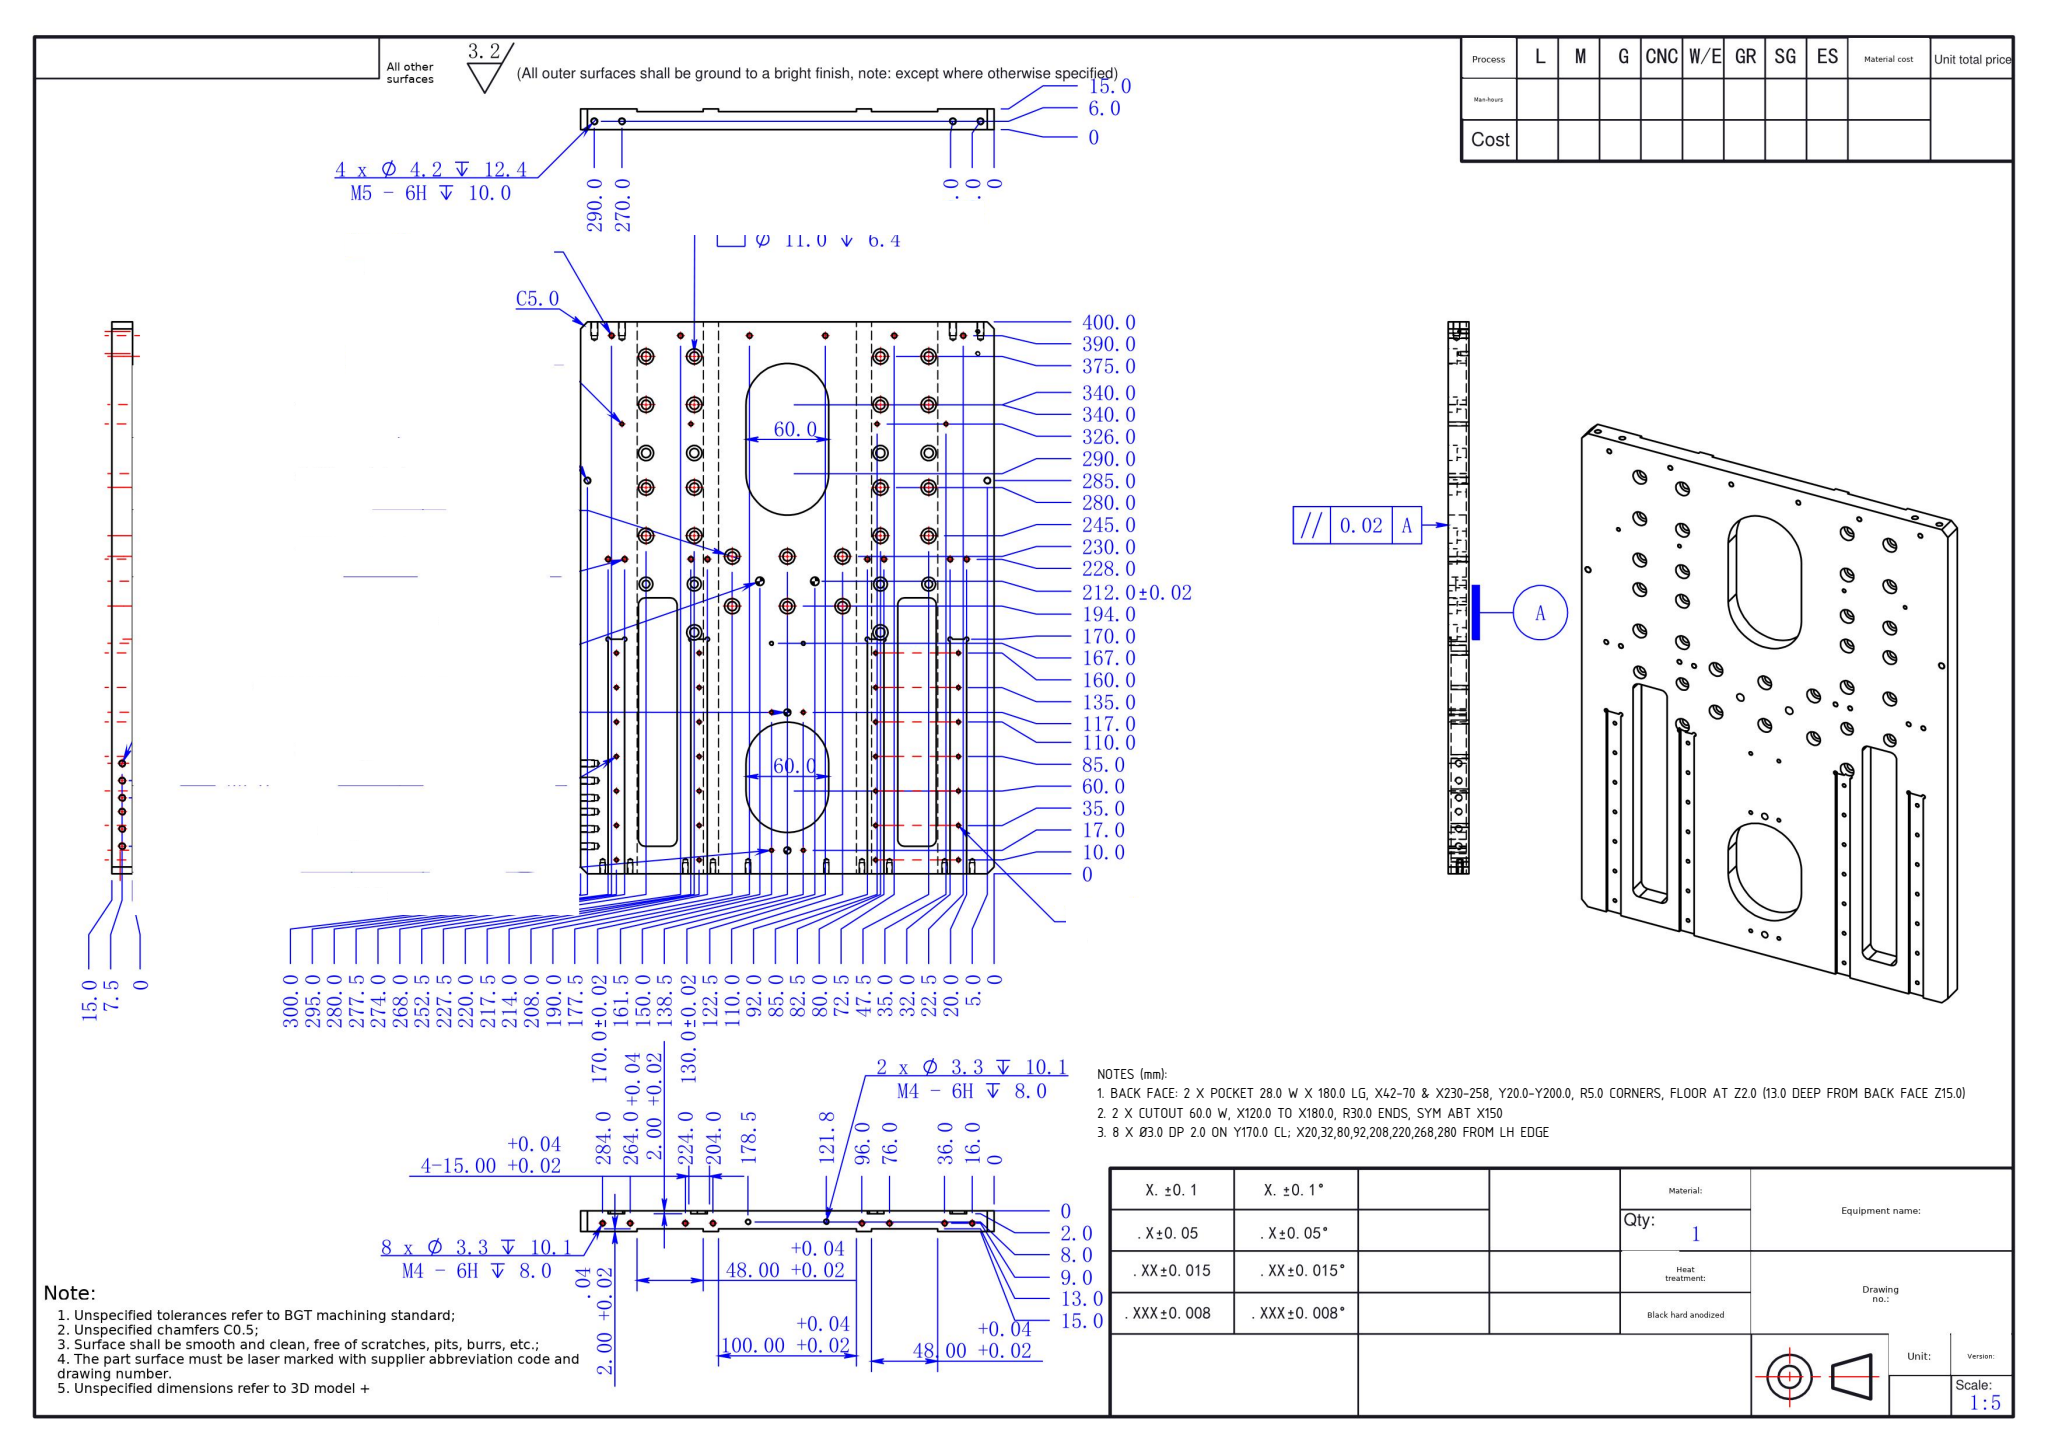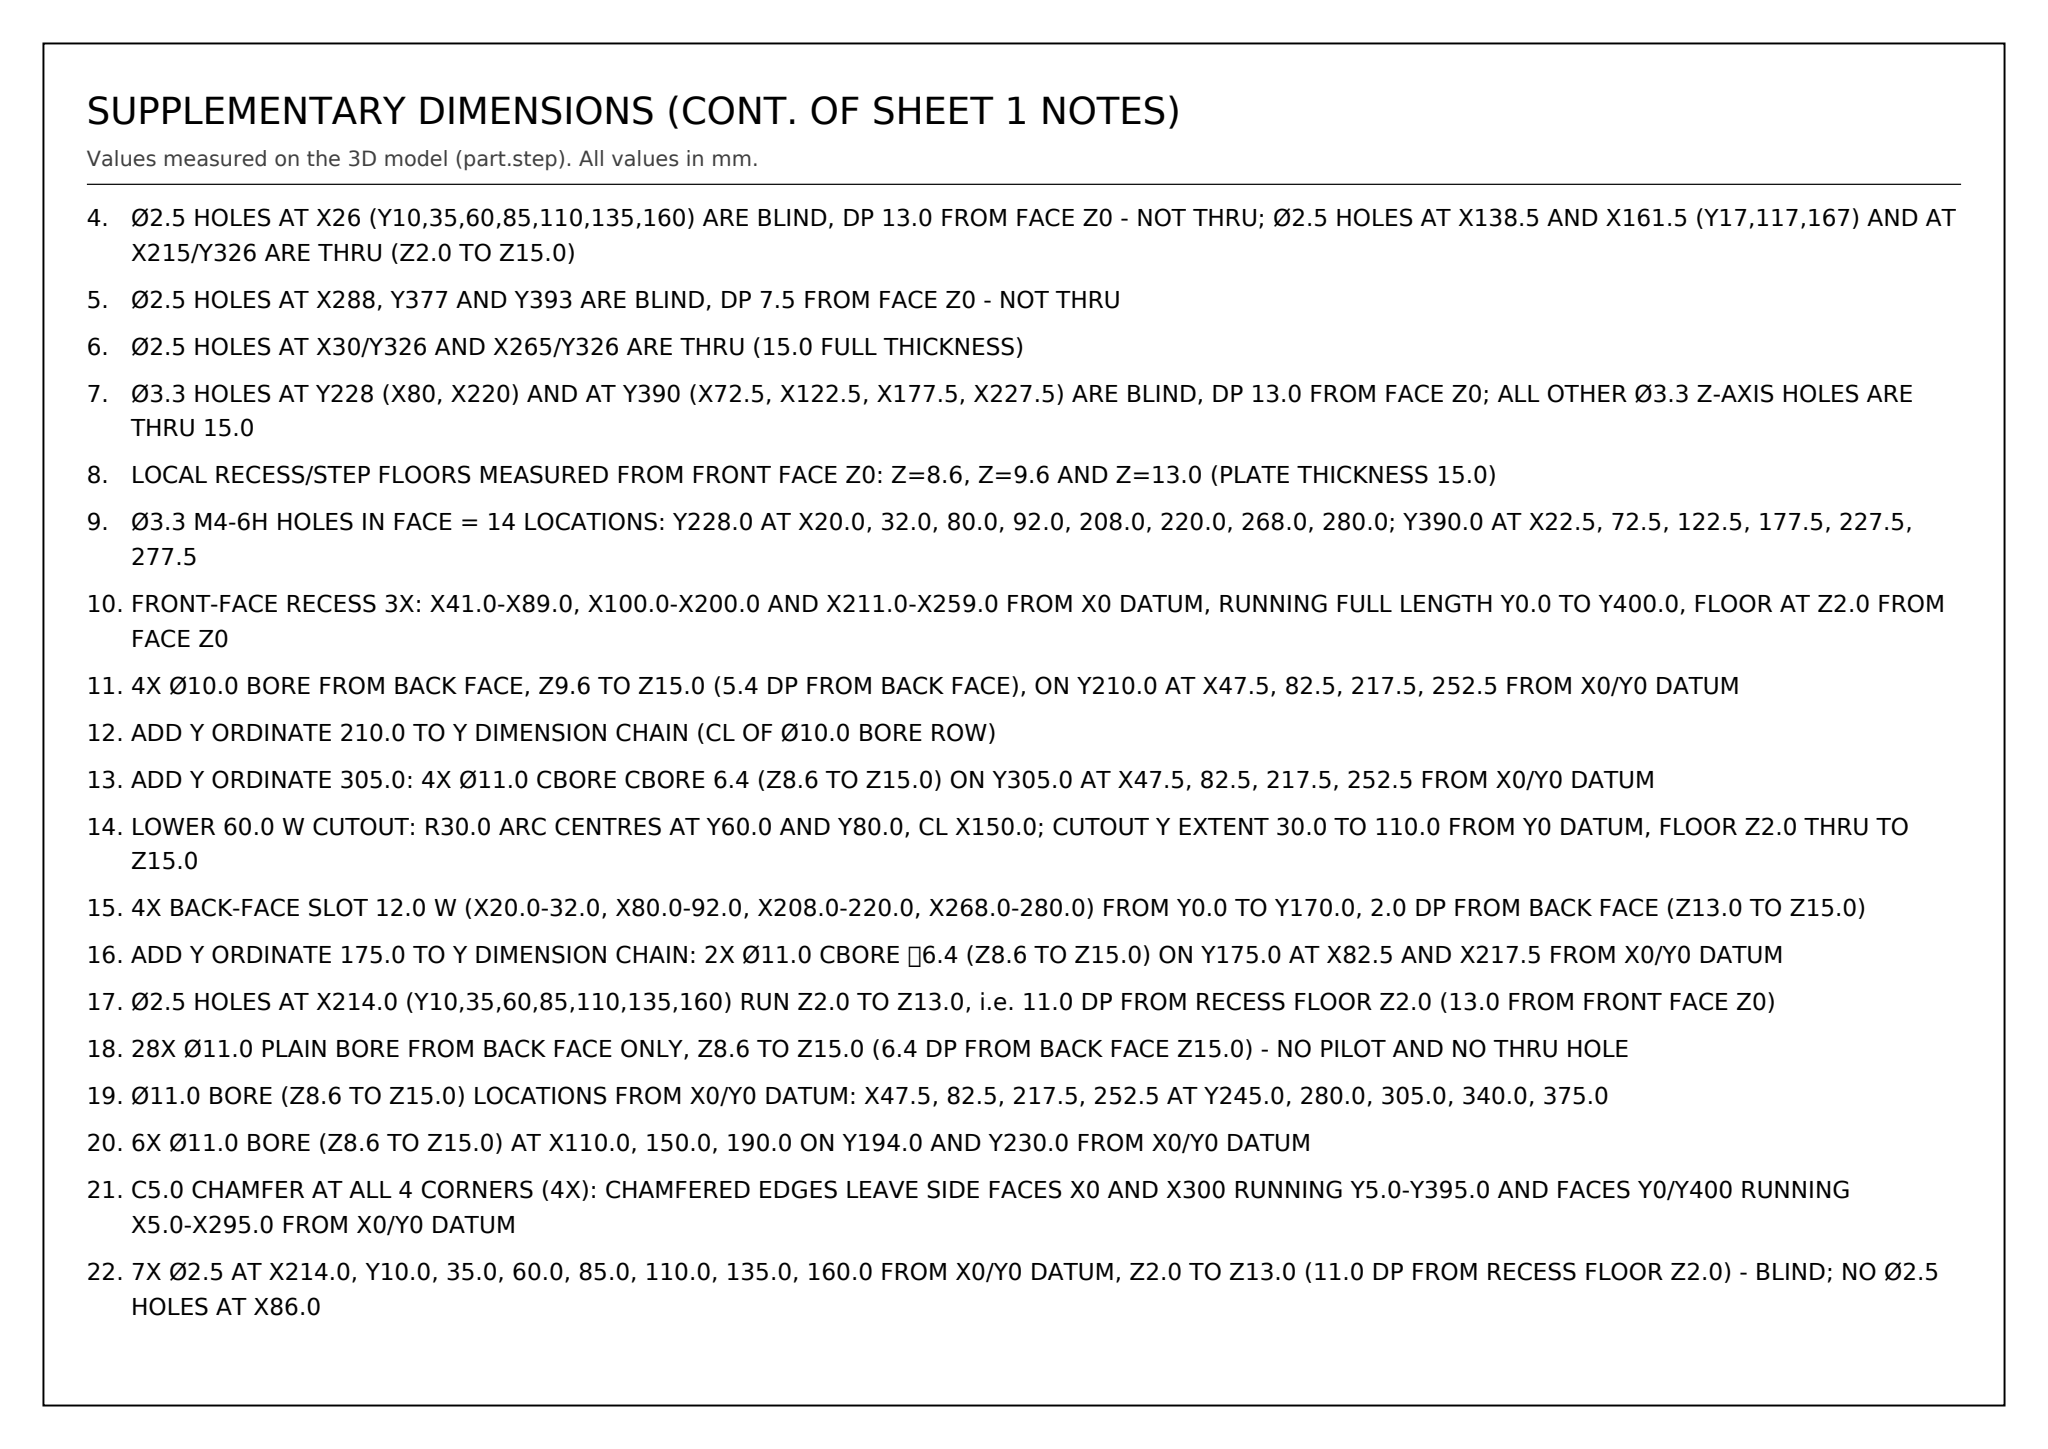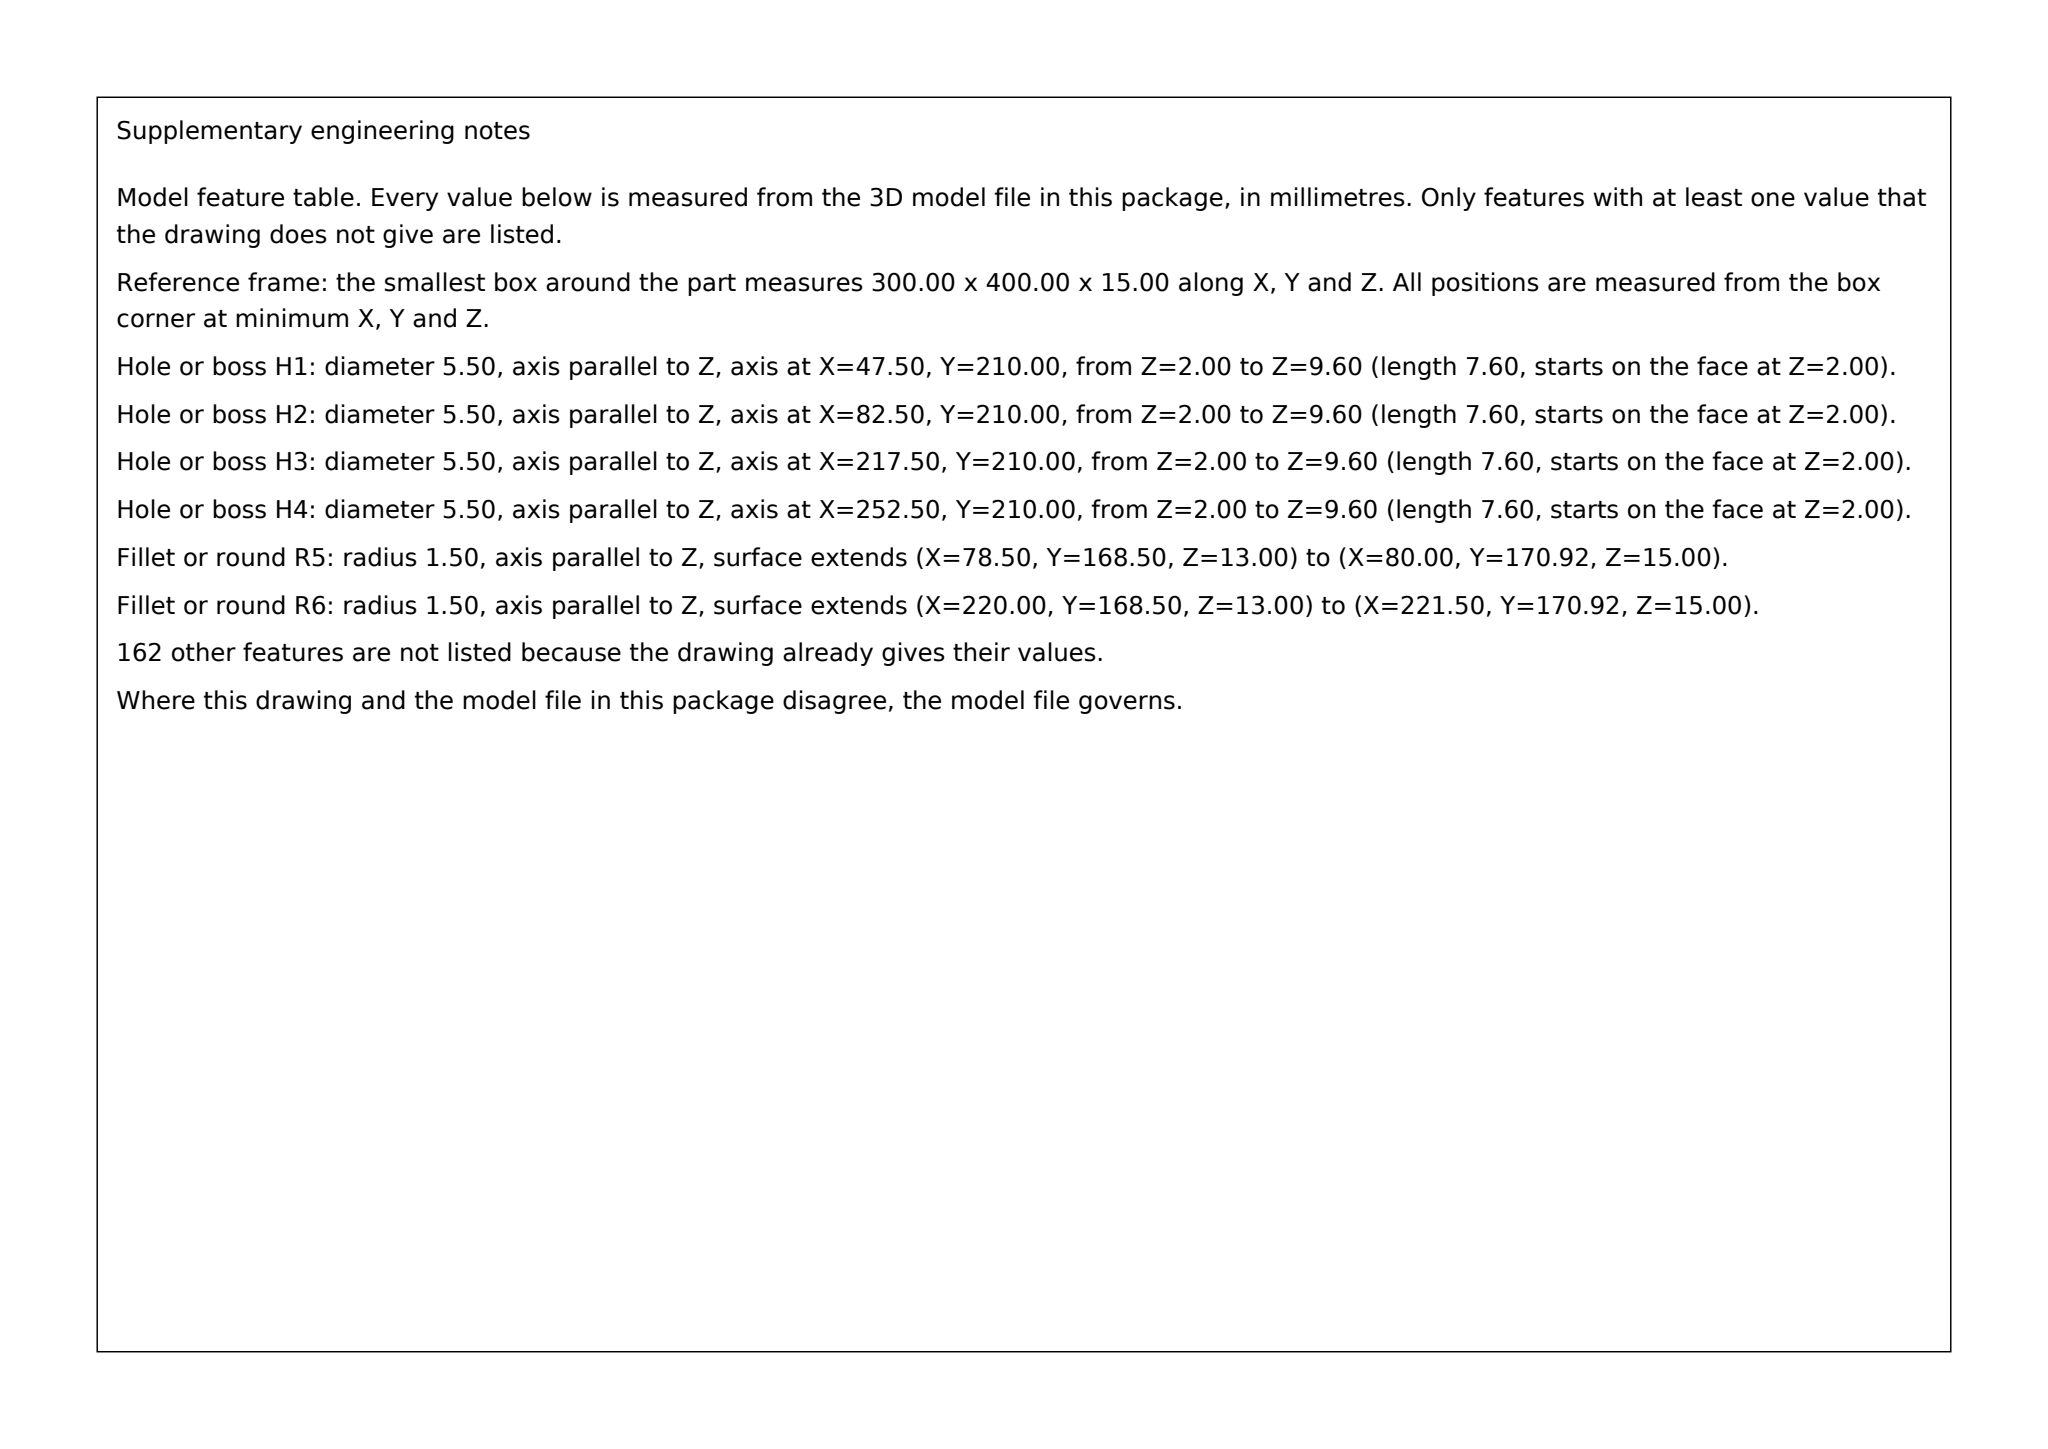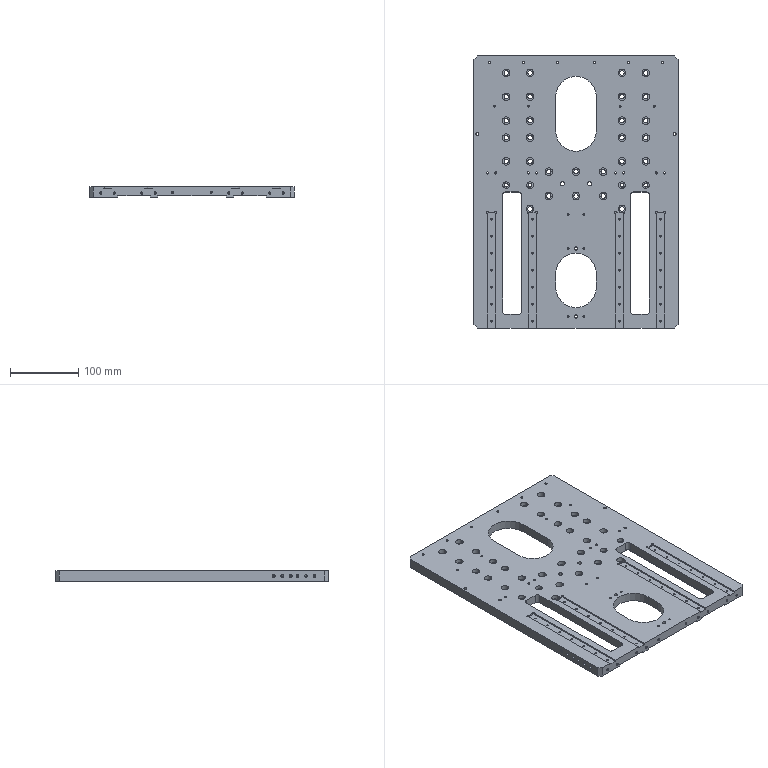Part | SolidWorks | mm | 1 solid | 438 faces | box 300 x 400 x 15 mm | volume 1333290 mm3 | cylinder 312 | plane 82 | cone 44 | commonest cylinder face diameters 2.5 x80 11 x56 6.6 x56 3.3 x48 4.2 x24 10 x16 3 x12 5.5 x8
Drawing notes:
BACK FACE: 2 X POCKET 28.0 W X 180.0 LG, X42-70 & X230-258, Y20.0-Y200.0, R5.0 CORNERS, FLOOR AT Z2.0 (13.0 DEEP FROM BACK FACE Z15.0) | from the solid: x-planes at 42.0, 70.0, 230.0, 258.0 (y 25.0-195.0, z 2.0-15.0) and y-planes at 20.0 & 200.0 (x 47-65 and 235-253, z 2.0-15.0); corner arcs are dia 10.0 (= R5.0) at (47,25),(47,195),(65,25),(65,195),(235,25),(235,195),(253,25),(253,195), z 2.0 to 15.0
2 X CUTOUT 60.0 W, X120.0 TO X180.0, R30.0 ENDS, SYM ABT X150 | from the solid: axis planes x=120.0 (2) and x=180.0 (2) = flats of two 60 wide cutouts, sym about X150
8 X Ø3.0 DP 2.0 ON Y170.0 CL; X20,32,80,92,208,220,268,280 FROM LH EDGE | from the solid: cylinders dia 3.0, axis z, y=170, len 2.0 at x=20,32,80,92,208,220,268,280 (8 holes)
Ø2.5 HOLES AT X26 (Y10,35,60,85,110,135,160) ARE BLIND, DP 13.0 FROM FACE Z0 - NOT THRU; Ø2.5 HOLES AT X138.5 AND X161.5 (Y17,117,167) AND AT X215/Y326 ARE THRU (Z2.0 TO Z15.0) | from the solid: hole/bore 2.5 z at [26.0,10/35/60/85/110/135/160] from 0.0 to 13.0 (blind); hole/bore 2.5 z at [138.5,17/117/167] and [161.5,17/117/167] from 2.0 to 15.0 (thru); hole/bore 2.5 z at [215.0,326.0] from 2.0 to 15.0 (thru)
Ø2.5 HOLES AT X288, Y377 AND Y393 ARE BLIND, DP 7.5 FROM FACE Z0 - NOT THRU | from the solid: cylinders [2.5,'z',[288.0,377.0/393.0,null],7.5,2]
Ø2.5 HOLES AT X30/Y326 AND X265/Y326 ARE THRU (15.0 FULL THICKNESS) | from the solid: cylinders [2.5,'z',[30.0/265.0,326.0,null],15.0,2]
Ø3.3 HOLES AT Y228 (X80, X220) AND AT Y390 (X72.5, X122.5, X177.5, X227.5) ARE BLIND, DP 13.0 FROM FACE Z0; ALL OTHER Ø3.3 Z-AXIS HOLES ARE THRU 15.0 | from the solid: cylinders [3.3,'z',...,13.0] vs [3.3,'z',...,15.0]
LOCAL RECESS/STEP FLOORS MEASURED FROM FRONT FACE Z0: Z=8.6, Z=9.6 AND Z=13.0 (PLATE THICKNESS 15.0) | from the solid: axis_planes ['z',8.6,28], ['z',9.6,4], ['z',13.0,4], ['z',15.0,1]
Ø3.3 M4-6H HOLES IN FACE = 14 LOCATIONS: Y228.0 AT X20.0, 32.0, 80.0, 92.0, 208.0, 220.0, 268.0, 280.0; Y390.0 AT X22.5, 72.5, 122.5, 177.5, 227.5, 277.5 | from the solid: cylinders dia 3.3 axis z, [x,y] positions
FRONT-FACE RECESS 3X: X41.0-X89.0, X100.0-X200.0 AND X211.0-X259.0 FROM X0 DATUM, RUNNING FULL LENGTH Y0.0 TO Y400.0, FLOOR AT Z2.0 FROM FACE Z0 | from the solid: x-planes at 41.0, 89.0, 100.0, 200.0, 211.0 and 259.0 each with extent y [0.0,400.0], z [0.0,2.0], area 800; holes at X138.5/X161.5 and X214 start at z 2.0 while holes at X26 start at z 0.0
4X Ø10.0 BORE FROM BACK FACE, Z9.6 TO Z15.0 (5.4 DP FROM BACK FACE), ON Y210.0 AT X47.5, 82.5, 217.5, 252.5 FROM X0/Y0 DATUM | from the solid: cylinders: hole/bore dia 10.0 axis z at (47.5,210),(82.5,210),(217.5,210),(252.5,210), from 9.6 to 15.0
ADD Y ORDINATE 210.0 TO Y DIMENSION CHAIN (CL OF Ø10.0 BORE ROW) | from the solid: cylinders: hole/bore dia 10.0 axis z at y=210.0 (X47.5, 82.5, 217.5, 252.5)
ADD Y ORDINATE 305.0: 4X Ø11.0 CBORE CBORE 6.4 (Z8.6 TO Z15.0) ON Y305.0 AT X47.5, 82.5, 217.5, 252.5 FROM X0/Y0 DATUM | from the solid: cylinders: hole/bore dia 11.0 axis z at (47.5,305),(82.5,305),(217.5,305),(252.5,305), from 8.6 to 15.0
LOWER 60.0 W CUTOUT: R30.0 ARC CENTRES AT Y60.0 AND Y80.0, CL X150.0; CUTOUT Y EXTENT 30.0 TO 110.0 FROM Y0 DATUM, FLOOR Z2.0 THRU TO Z15.0 | from the solid: cylinders: concave arc dia 60.0 axis z at (150,60) and (150,80), from 2.0 to 15.0, 180 deg each
4X BACK-FACE SLOT 12.0 W (X20.0-32.0, X80.0-92.0, X208.0-220.0, X268.0-280.0) FROM Y0.0 TO Y170.0, 2.0 DP FROM BACK FACE (Z13.0 TO Z15.0) | from the solid: axis_planes: x=20/32/80/92/208/220/268/280 with y extent [0.0,168.5], z extent [13.0,15.0]
ADD Y ORDINATE 175.0 TO Y DIMENSION CHAIN: 2X Ø11.0 CBORE ⍄6.4 (Z8.6 TO Z15.0) ON Y175.0 AT X82.5 AND X217.5 FROM X0/Y0 DATUM | from the solid: cylinders: hole/bore dia 11.0, axis z at (82.5,175.0) and (217.5,175.0), from Z8.6 to Z15.0
Ø2.5 HOLES AT X214.0 (Y10,35,60,85,110,135,160) RUN Z2.0 TO Z13.0, i.e. 11.0 DP FROM RECESS FLOOR Z2.0 (13.0 FROM FRONT FACE Z0) | from the solid: cylinders: hole/bore dia 2.5 axis z at [214.0,10.0 ...160.0], from 2.0 to 13.0
28X Ø11.0 PLAIN BORE FROM BACK FACE ONLY, Z8.6 TO Z15.0 (6.4 DP FROM BACK FACE Z15.0) - NO PILOT AND NO THRU HOLE | from the solid: cylinders kind hole/bore dia 11.0 axis z, from 8.6 to 15.0 (28 occurrences)
Ø11.0 BORE (Z8.6 TO Z15.0) LOCATIONS FROM X0/Y0 DATUM: X47.5, 82.5, 217.5, 252.5 AT Y245.0, 280.0, 305.0, 340.0, 375.0 | from the solid: cylinders dia 11.0 axis z at (47.5/82.5/217.5/252.5, 245/280/305/340/375), from 8.6 to 15.0
6X Ø11.0 BORE (Z8.6 TO Z15.0) AT X110.0, 150.0, 190.0 ON Y194.0 AND Y230.0 FROM X0/Y0 DATUM | from the solid: cylinders dia 11.0 axis z at [110/150/190, 194.0] and [110/150/190, 230.0], from 8.6 to 15.0
C5.0 CHAMFER AT ALL 4 CORNERS (4X): CHAMFERED EDGES LEAVE SIDE FACES X0 AND X300 RUNNING Y5.0-Y395.0 AND FACES Y0/Y400 RUNNING X5.0-X295.0 FROM X0/Y0 DATUM | from the solid: axis_planes: x=0.0 extent y[5.0,395.0]; x=300.0 extent y[5.0,395.0]; y=0.0 extent x[5.0,295.0] (bbox 300.0 x 400.0 x 15.0)
7X Ø2.5 AT X214.0, Y10.0, 35.0, 60.0, 85.0, 110.0, 135.0, 160.0 FROM X0/Y0 DATUM, Z2.0 TO Z13.0 (11.0 DP FROM RECESS FLOOR Z2.0) - BLIND; NO Ø2.5 HOLES AT X86.0 | from the solid: cylinders hole/bore Ø2.5 z-axis at (214.0, 10/35/60/85/110/135/160) from 2.0 to 13.0; no Ø2.5 cylinder at X86.0 in model
build123d program:
from build123d import *

# Parameters (mm, degrees)
SKETCH1_W                                       = 300
SKETCH1_H                                       = 285
BOSS_EXTRUDE1_DEPTH                             = 15
SKETCH2_W                                       = 300
SKETCH2_H                                       = 15
BOSS_EXTRUDE2_DEPTH                             = 115
CHAMFER2_SIZE                                   = 5
SKETCH4_W                                       = 12
SKETCH4_H                                       = 2
CUT_EXTRUDE2_DEPTH                              = 170
SKETCH5_R                                       = 1.5
CUT_EXTRUDE3_DEPTH                              = 2
SKETCH6_W                                       = 48
SKETCH6_H                                       = 2
CUT_EXTRUDE4_DEPTH                              = 428.463
SKETCH7_W                                       = 100
SKETCH7_H                                       = 2
CUT_EXTRUDE5_DEPTH                              = 428.463
SKETCH8_R                                       = 30
CUT_EXTRUDE6_DEPTH                              = 299.287
M6_HEX_SOCKET_HEAD_CAP_SCREW_CBORE1_D           = 6.6
M6_HEX_SOCKET_HEAD_CAP_SCREW_CBORE1_CBORE_D     = 11
M6_HEX_SOCKET_HEAD_CAP_SCREW_CBORE1_CBORE_DEPTH = 6.4
M6_HEX_SOCKET_HEAD_CAP_SCREW_CBORE2_D           = 6.6
M6_HEX_SOCKET_HEAD_CAP_SCREW_CBORE2_CBORE_D     = 11
M6_HEX_SOCKET_HEAD_CAP_SCREW_CBORE2_CBORE_DEPTH = 6.4
M4_TAPPED_HOLE1_D                               = 3.3
M4_TAPPED_HOLE1_DEPTH                           = 10.1
M4_TAPPED_HOLE1_TIP                             = 0.9914
SIZE_MM_DOWEL_PIN_HOLE_1_D                      = 6
CUT_EXTRUDE7_DEPTH                              = 299.381
CUT_EXTRUDE8_DEPTH                              = 299.381
M3_TAPPED_HOLE1_D                               = 2.5
M3_TAPPED_HOLE2_D                               = 2.5
M3_TAPPED_HOLE2_DEPTH                           = 7.5
M3_TAPPED_HOLE2_TIP                             = 0.7511
M4_TAPPED_HOLE3_D                               = 3.3
M3_TAPPED_HOLE3_D                               = 2.5
LPATTERN1_COUNT                                 = 2
LPATTERN1_PITCH                                 = 60
MIRROR3_COPY_1_D                                = 2.5
M4_TAPPED_HOLE2_D                               = 3.3
M3_TAPPED_HOLE4_D                               = 2.5
SIZE_MM_DOWEL_PIN_HOLE_2_D                      = 5
SKETCH35_W                                      = 28
SKETCH35_H                                      = 180
CUT_EXTRUDE9_DEPTH                              = 299.381
FILLET2_R                                       = 5
M5_TAPPED_HOLE1_D                               = 4.2
M5_TAPPED_HOLE1_DEPTH                           = 12.4
M5_TAPPED_HOLE1_TIP                             = 1.262
M5_HEX_SOCKET_HEAD_CAP_SCREW_CBORE2_D           = 5.5
M5_HEX_SOCKET_HEAD_CAP_SCREW_CBORE2_CBORE_D     = 10
M5_HEX_SOCKET_HEAD_CAP_SCREW_CBORE2_CBORE_DEPTH = 5.4
M6_HEX_SOCKET_HEAD_CAP_SCREW_CBORE3_D           = 6.6
M6_HEX_SOCKET_HEAD_CAP_SCREW_CBORE3_CBORE_D     = 11
M6_HEX_SOCKET_HEAD_CAP_SCREW_CBORE3_CBORE_DEPTH = 6.4
M4_TAPPED_HOLE4_D                               = 3.3
M4_TAPPED_HOLE4_DEPTH                           = 10.1
M4_TAPPED_HOLE4_TIP                             = 0.9914
M5_TAPPED_HOLE2_D                               = 4.2
M5_TAPPED_HOLE2_DEPTH                           = 12.4
M5_TAPPED_HOLE2_TIP                             = 1.262
M5_TAPPED_HOLE3_D                               = 4.2


with BuildPart() as part:
    # Sketch1 → Boss-Extrude1 (new body)
    with BuildSketch(Plane.XY):
        Rectangle(SKETCH1_W, SKETCH1_H)
    extrude(amount=BOSS_EXTRUDE1_DEPTH)

    # Sketch2 → Boss-Extrude2 (add)
    with BuildSketch(Plane(origin=(0, 142.5, 0), x_dir=(1, 0, 0), z_dir=(0, 1, 0))):
        with Locations((0, -7.5)):
            Rectangle(SKETCH2_W, SKETCH2_H)
    extrude(amount=BOSS_EXTRUDE2_DEPTH)

    # Chamfer2
    chamfer2_edges = [part.edges().sort_by_distance(p)[0] for p in [
        (150, 257.5, 7.5),
        (-150, 257.5, 7.5),
        (150, -142.5, 7.5),
        (-150, -142.5, 7.5),
    ]]
    chamfer(chamfer2_edges, length=CHAMFER2_SIZE)

    # Sketch4 → Cut-Extrude2 (cut)
    with BuildSketch(Plane.XZ.offset(142.5)):
        with Locations((-124, 14)):
            Rectangle(SKETCH4_W, SKETCH4_H)
        with Locations((-64, 14)):
            Rectangle(SKETCH4_W, SKETCH4_H)
    cut_extrude2 = extrude(amount=-CUT_EXTRUDE2_DEPTH, mode=Mode.SUBTRACT)

    # Sketch5 → Cut-Extrude3 (cut)
    with BuildSketch(Plane.XY.offset(15)):
        with Locations((-130, 27.5)):
            Circle(SKETCH5_R)
        with Locations((-118, 27.5)):
            Circle(SKETCH5_R)
        with Locations((-70, 27.5)):
            Circle(SKETCH5_R)
        with Locations((-58, 27.5)):
            Circle(SKETCH5_R)
    cut_extrude3 = extrude(amount=-CUT_EXTRUDE3_DEPTH, mode=Mode.SUBTRACT)

    # Mirror1: Cut-Extrude2, Cut-Extrude3 across plane
    add(cut_extrude2.mirror(Plane.ZY), mode=Mode.SUBTRACT)
    add(cut_extrude3.mirror(Plane.ZY), mode=Mode.SUBTRACT)

    # Sketch6 → Cut-Extrude4 (cut, through all)
    with BuildSketch(Plane(origin=(0, 257.5, 0), x_dir=(1, 0, 0), z_dir=(0, 1, 0))):
        with Locations((85, -1)):
            Rectangle(SKETCH6_W, SKETCH6_H)
        with Locations((-85, -1)):
            Rectangle(SKETCH6_W, SKETCH6_H)
    extrude(amount=-CUT_EXTRUDE4_DEPTH, mode=Mode.SUBTRACT)

    # Sketch7 → Cut-Extrude5 (cut, through all)
    with BuildSketch(Plane(origin=(0, 257.5, 0), x_dir=(1, 0, 0), z_dir=(0, 1, 0))):
        with Locations((0, -1)):
            Rectangle(SKETCH7_W, SKETCH7_H)
    extrude(amount=-CUT_EXTRUDE5_DEPTH, mode=Mode.SUBTRACT)

    # Sketch8 → Cut-Extrude6 (cut, through all)
    with BuildSketch(Plane(origin=(0, 0, 2), x_dir=(-1, 0, 0), z_dir=(0, 0, -1))):
        with Locations((0, 197.5)):
            Circle(SKETCH8_R)
        with Locations((0, -82.5)):
            Circle(SKETCH8_R)
    extrude(amount=-CUT_EXTRUDE6_DEPTH, mode=Mode.SUBTRACT)

    # M6 Hex Socket Head Cap Screw CBORE1 (through all)
    with Locations(Plane.XY.offset(15)):
        with Locations((-40, 87.5), (40, 87.5), (-40, 51.5), (40, 51.5), (0, 87.5), (0, 51.5)):
            CounterBoreHole(M6_HEX_SOCKET_HEAD_CAP_SCREW_CBORE1_D / 2, M6_HEX_SOCKET_HEAD_CAP_SCREW_CBORE1_CBORE_D / 2, M6_HEX_SOCKET_HEAD_CAP_SCREW_CBORE1_CBORE_DEPTH)

    # M6 Hex Socket Head Cap Screw CBORE2 (through all)
    with Locations(Plane.XY.offset(15)):
        with Locations((102.5, 232.5), (67.5, 232.5), (67.5, 197.5), (102.5, 197.5), (67.5, 137.5), (102.5, 137.5), (67.5, 102.5), (102.5, 102.5)):
            m6_hex_socket_head_cap_screw_cbore2 = CounterBoreHole(M6_HEX_SOCKET_HEAD_CAP_SCREW_CBORE2_D / 2, M6_HEX_SOCKET_HEAD_CAP_SCREW_CBORE2_CBORE_D / 2, M6_HEX_SOCKET_HEAD_CAP_SCREW_CBORE2_CBORE_DEPTH)

    # Mirror2: M6 Hex Socket Head Cap Screw CBORE2 across plane
    add(m6_hex_socket_head_cap_screw_cbore2.mirror(Plane(origin=(0, 0, 0), x_dir=(0, 0, 1), z_dir=(1, 0, 0))), mode=Mode.SUBTRACT)

    # M4 Tapped Hole1
    with Locations(Plane(origin=(0, -142.5, 0), x_dir=(-1, 0, 0), z_dir=(0, -1, 0))):
        with Locations((134, -6), (114, -6), (74, -6), (54, -6), (-54, -6), (-74, -6), (-114, -6), (-134, -6)):
            Hole(M4_TAPPED_HOLE1_D / 2, depth=M4_TAPPED_HOLE1_DEPTH)
            with Locations((0, 0, -(M4_TAPPED_HOLE1_DEPTH + M4_TAPPED_HOLE1_TIP / 2))):  # 118° drill point
                Cone(0, M4_TAPPED_HOLE1_D / 2, M4_TAPPED_HOLE1_TIP, mode=Mode.SUBTRACT)

    # Size mm Dowel Pin Hole 1 (through all)
    with Locations(Plane.XY.offset(15)):
        with Locations((-20, 69.5), (20, 69.5)):
            Hole(SIZE_MM_DOWEL_PIN_HOLE_1_D / 2)

    # Sketch19 → Cut-Extrude7 (cut, through all)
    with BuildSketch(Plane.XY.offset(15)):
        with BuildLine():
            Line((30, 197.5), (30, 147.5))
            ThreePointArc((30, 147.5), (0, 117.5), (-30, 147.5))
            Line((-30, 147.5), (-30, 197.5))
            ThreePointArc((-30, 197.5), (0, 227.5), (30, 197.5))
        make_face()
    extrude(amount=-CUT_EXTRUDE7_DEPTH, mode=Mode.SUBTRACT)

    # Sketch20 → Cut-Extrude8 (cut, through all)
    with BuildSketch(Plane.XY.offset(15)):
        with BuildLine():
            Line((-30, -82.5), (-30, -62.5))
            ThreePointArc((-30, -62.5), (0, -32.5), (30, -62.5))
            Line((30, -62.5), (30, -82.5))
            ThreePointArc((30, -82.5), (0, -112.5), (-30, -82.5))
        make_face()
    extrude(amount=-CUT_EXTRUDE8_DEPTH, mode=Mode.SUBTRACT)

    # M3 Tapped Hole1 (through all)
    with Locations(Plane.XY.offset(15)):
        with Locations((11.5, -125.5), (-11.5, -125.5), (-11.5, -25.5), (11.5, -25.5), (-11.5, 24.5), (11.5, 24.5)):
            Hole(M3_TAPPED_HOLE1_D / 2)

    # M3 Tapped Hole2
    with Locations(Plane(origin=(0, 0, 0), x_dir=(-1, 0, 0), z_dir=(0, 0, -1))):
        with Locations((-138, 250.5), (-138, 234.5)):
            Hole(M3_TAPPED_HOLE2_D / 2, depth=M3_TAPPED_HOLE2_DEPTH)
            with Locations((0, 0, -(M3_TAPPED_HOLE2_DEPTH + M3_TAPPED_HOLE2_TIP / 2))):  # 118° drill point
                Cone(0, M3_TAPPED_HOLE2_D / 2, M3_TAPPED_HOLE2_TIP, mode=Mode.SUBTRACT)

    # M4 Tapped Hole3 (through all)
    with Locations(Plane.XY.offset(15)):
        with Locations((-127.5, 247.5), (-77.5, 247.5), (-27.5, 247.5), (27.5, 247.5), (77.5, 247.5), (127.5, 247.5)):
            Hole(M4_TAPPED_HOLE3_D / 2)

    # M3 Tapped Hole3 (through all)
    with Locations(Plane.XY.offset(13)):
        with Locations((124, -132.5), (124, -107.5), (124, -82.5), (124, -57.5), (124, -32.5), (124, -7.5), (124, 17.5)):
            m3_tapped_hole3 = Hole(M3_TAPPED_HOLE3_D / 2)

    # LPattern1: M3 Tapped Hole3 ×2
    with Locations(*[(-i * LPATTERN1_PITCH, 0, 0) for i in range(1, LPATTERN1_COUNT)]):
        add(m3_tapped_hole3, mode=Mode.SUBTRACT)

    # Mirror3: M3 Tapped Hole3 across plane
    add(m3_tapped_hole3.mirror(Plane(origin=(0, 0, 0), x_dir=(0, 0, 1), z_dir=(1, 0, 0))), mode=Mode.SUBTRACT)

    # Mirror3 copy 1 (through all)
    with Locations(Plane(origin=(60, 0, 13), x_dir=(-1, 0, 0), z_dir=(0, 0, 1))):
        with Locations((124, 132.5), (124, 107.5), (124, 82.5), (124, 57.5), (124, 32.5), (124, 7.5), (124, -17.5)):
            Hole(MIRROR3_COPY_1_D / 2)

    # M4 Tapped Hole2 (through all)
    with Locations(Plane.XY.offset(15)):
        with Locations((-130, 85.5), (-118, 85.5), (-70, 85.5), (-58, 85.5), (58, 85.5), (70, 85.5), (118, 85.5), (130, 85.5)):
            Hole(M4_TAPPED_HOLE2_D / 2)

    # M3 Tapped Hole4 (through all)
    with Locations(Plane.XY.offset(15)):
        with Locations((65, 183.5), (115, 183.5), (-120, 183.5), (-70, 183.5)):
            Hole(M3_TAPPED_HOLE4_D / 2)

    # Size mm Dowel Pin Hole 2 (through all)
    with Locations(Plane.XY.offset(15)):
        with Locations((0, -125.5), (0, -25.5)):
            Hole(SIZE_MM_DOWEL_PIN_HOLE_2_D / 2)

    # Sketch35 → Cut-Extrude9 (cut, through all)
    with BuildSketch(Plane.XY.offset(15)):
        with Locations((-94, -32.5)):
            Rectangle(SKETCH35_W, SKETCH35_H)
        with Locations((94, -32.5)):
            Rectangle(SKETCH35_W, SKETCH35_H)
    extrude(amount=-CUT_EXTRUDE9_DEPTH, mode=Mode.SUBTRACT)

    # Fillet2
    fillet2_edges = [part.edges().sort_by_distance(p)[0] for p in [
        (-108, -122.5, 8.5),
        (-108, 57.5, 8.5),
        (-80, 57.5, 8.5),
        (-80, -122.5, 8.5),
        (80, -122.5, 8.5),
        (80, 57.5, 8.5),
        (108, 57.5, 8.5),
        (108, -122.5, 8.5),
    ]]
    fillet(fillet2_edges, radius=FILLET2_R)

    # M5 Tapped Hole1
    with Locations(Plane.ZY.offset(150)):
        with Locations((7.5, -122.5), (7.5, -97.5), (7.5, -110), (7.5, -87.5), (7.5, -75), (7.5, -62.5)):
            Hole(M5_TAPPED_HOLE1_D / 2, depth=M5_TAPPED_HOLE1_DEPTH)
            with Locations((0, 0, -(M5_TAPPED_HOLE1_DEPTH + M5_TAPPED_HOLE1_TIP / 2))):  # 118° drill point
                Cone(0, M5_TAPPED_HOLE1_D / 2, M5_TAPPED_HOLE1_TIP, mode=Mode.SUBTRACT)

    # M5 Hex Socket Head Cap Screw CBORE2 (through all)
    with Locations(Plane.XY.offset(15)):
        with Locations((-102.5, 67.5), (-67.5, 67.5), (67.5, 67.5), (102.5, 67.5)):
            CounterBoreHole(M5_HEX_SOCKET_HEAD_CAP_SCREW_CBORE2_D / 2, M5_HEX_SOCKET_HEAD_CAP_SCREW_CBORE2_CBORE_D / 2, M5_HEX_SOCKET_HEAD_CAP_SCREW_CBORE2_CBORE_DEPTH)

    # M6 Hex Socket Head Cap Screw CBORE3 (through all)
    with Locations(Plane.XY.offset(15)):
        with Locations((67.5, 162.5), (102.5, 162.5), (-102.5, 162.5), (-67.5, 162.5), (-67.5, 32.5), (67.5, 32.5)):
            CounterBoreHole(M6_HEX_SOCKET_HEAD_CAP_SCREW_CBORE3_D / 2, M6_HEX_SOCKET_HEAD_CAP_SCREW_CBORE3_CBORE_D / 2, M6_HEX_SOCKET_HEAD_CAP_SCREW_CBORE3_CBORE_DEPTH)

    # M4 Tapped Hole4
    with Locations(Plane(origin=(0, -142.5, 0), x_dir=(-1, 0, 0), z_dir=(0, -1, 0))):
        with Locations((-28.221, -7.169), (28.5, -7)):
            Hole(M4_TAPPED_HOLE4_D / 2, depth=M4_TAPPED_HOLE4_DEPTH)
            with Locations((0, 0, -(M4_TAPPED_HOLE4_DEPTH + M4_TAPPED_HOLE4_TIP / 2))):  # 118° drill point
                Cone(0, M4_TAPPED_HOLE4_D / 2, M4_TAPPED_HOLE4_TIP, mode=Mode.SUBTRACT)

    # M5 Tapped Hole2
    with Locations(Plane(origin=(0, 257.5, 0), x_dir=(1, 0, 0), z_dir=(0, 1, 0))):
        with Locations((-140, -9), (-120, -9), (120, -9), (140, -9)):
            Hole(M5_TAPPED_HOLE2_D / 2, depth=M5_TAPPED_HOLE2_DEPTH)
            with Locations((0, 0, -(M5_TAPPED_HOLE2_DEPTH + M5_TAPPED_HOLE2_TIP / 2))):  # 118° drill point
                Cone(0, M5_TAPPED_HOLE2_D / 2, M5_TAPPED_HOLE2_TIP, mode=Mode.SUBTRACT)

    # M5 Tapped Hole3 (through all)
    with Locations(Plane.XY.offset(15)):
        with Locations((145, 142.5), (-145, 142.5)):
            Hole(M5_TAPPED_HOLE3_D / 2)


solid = part.part